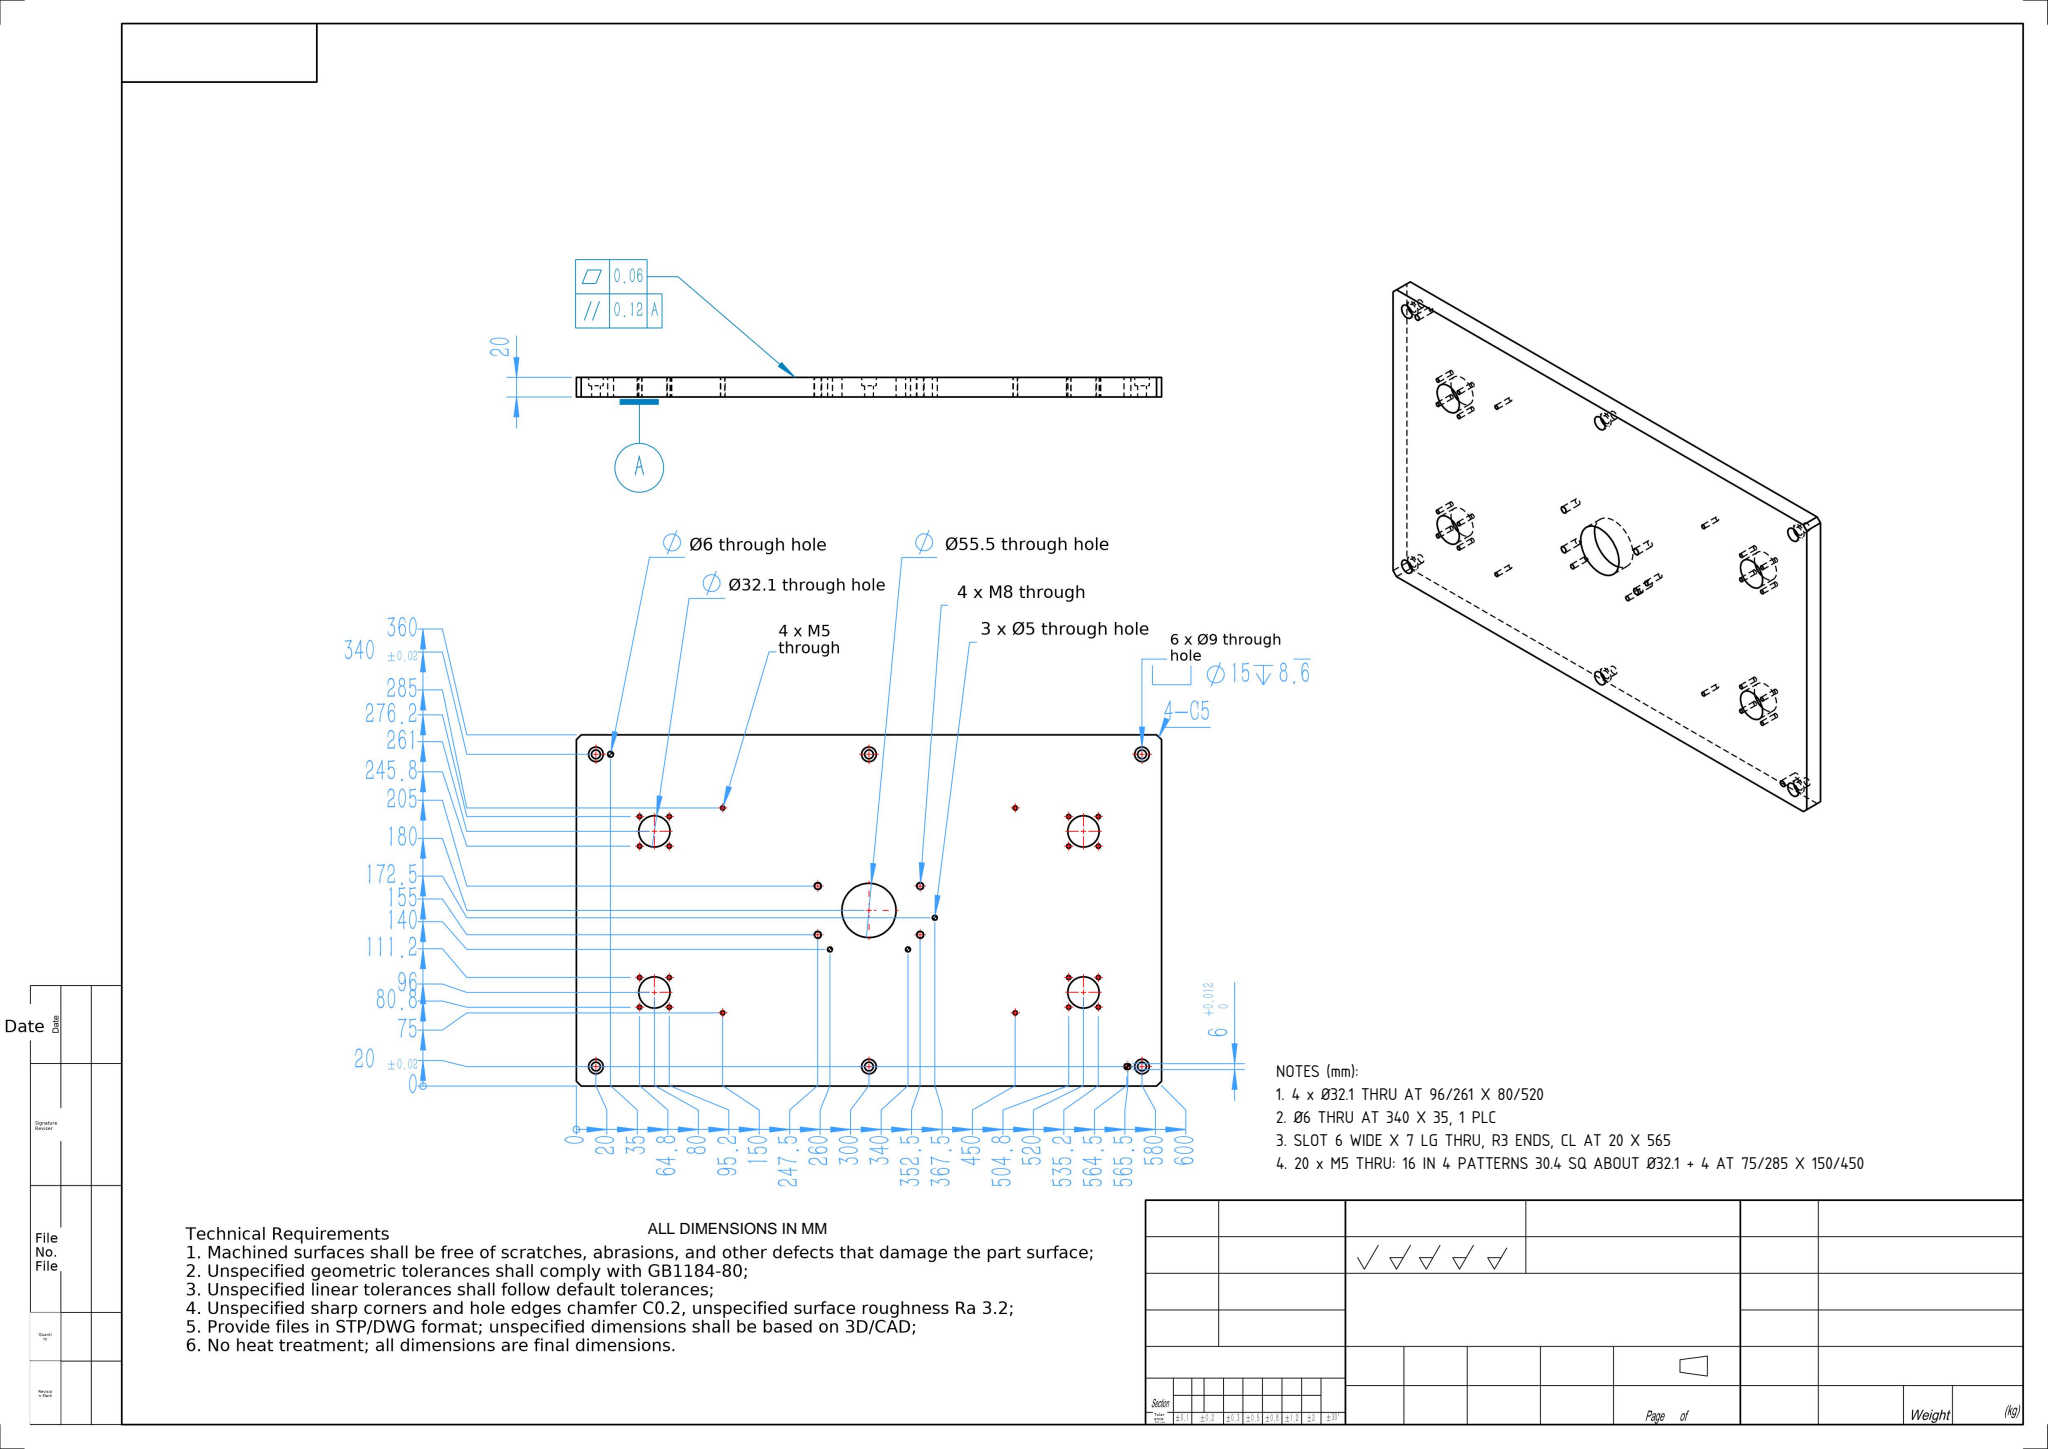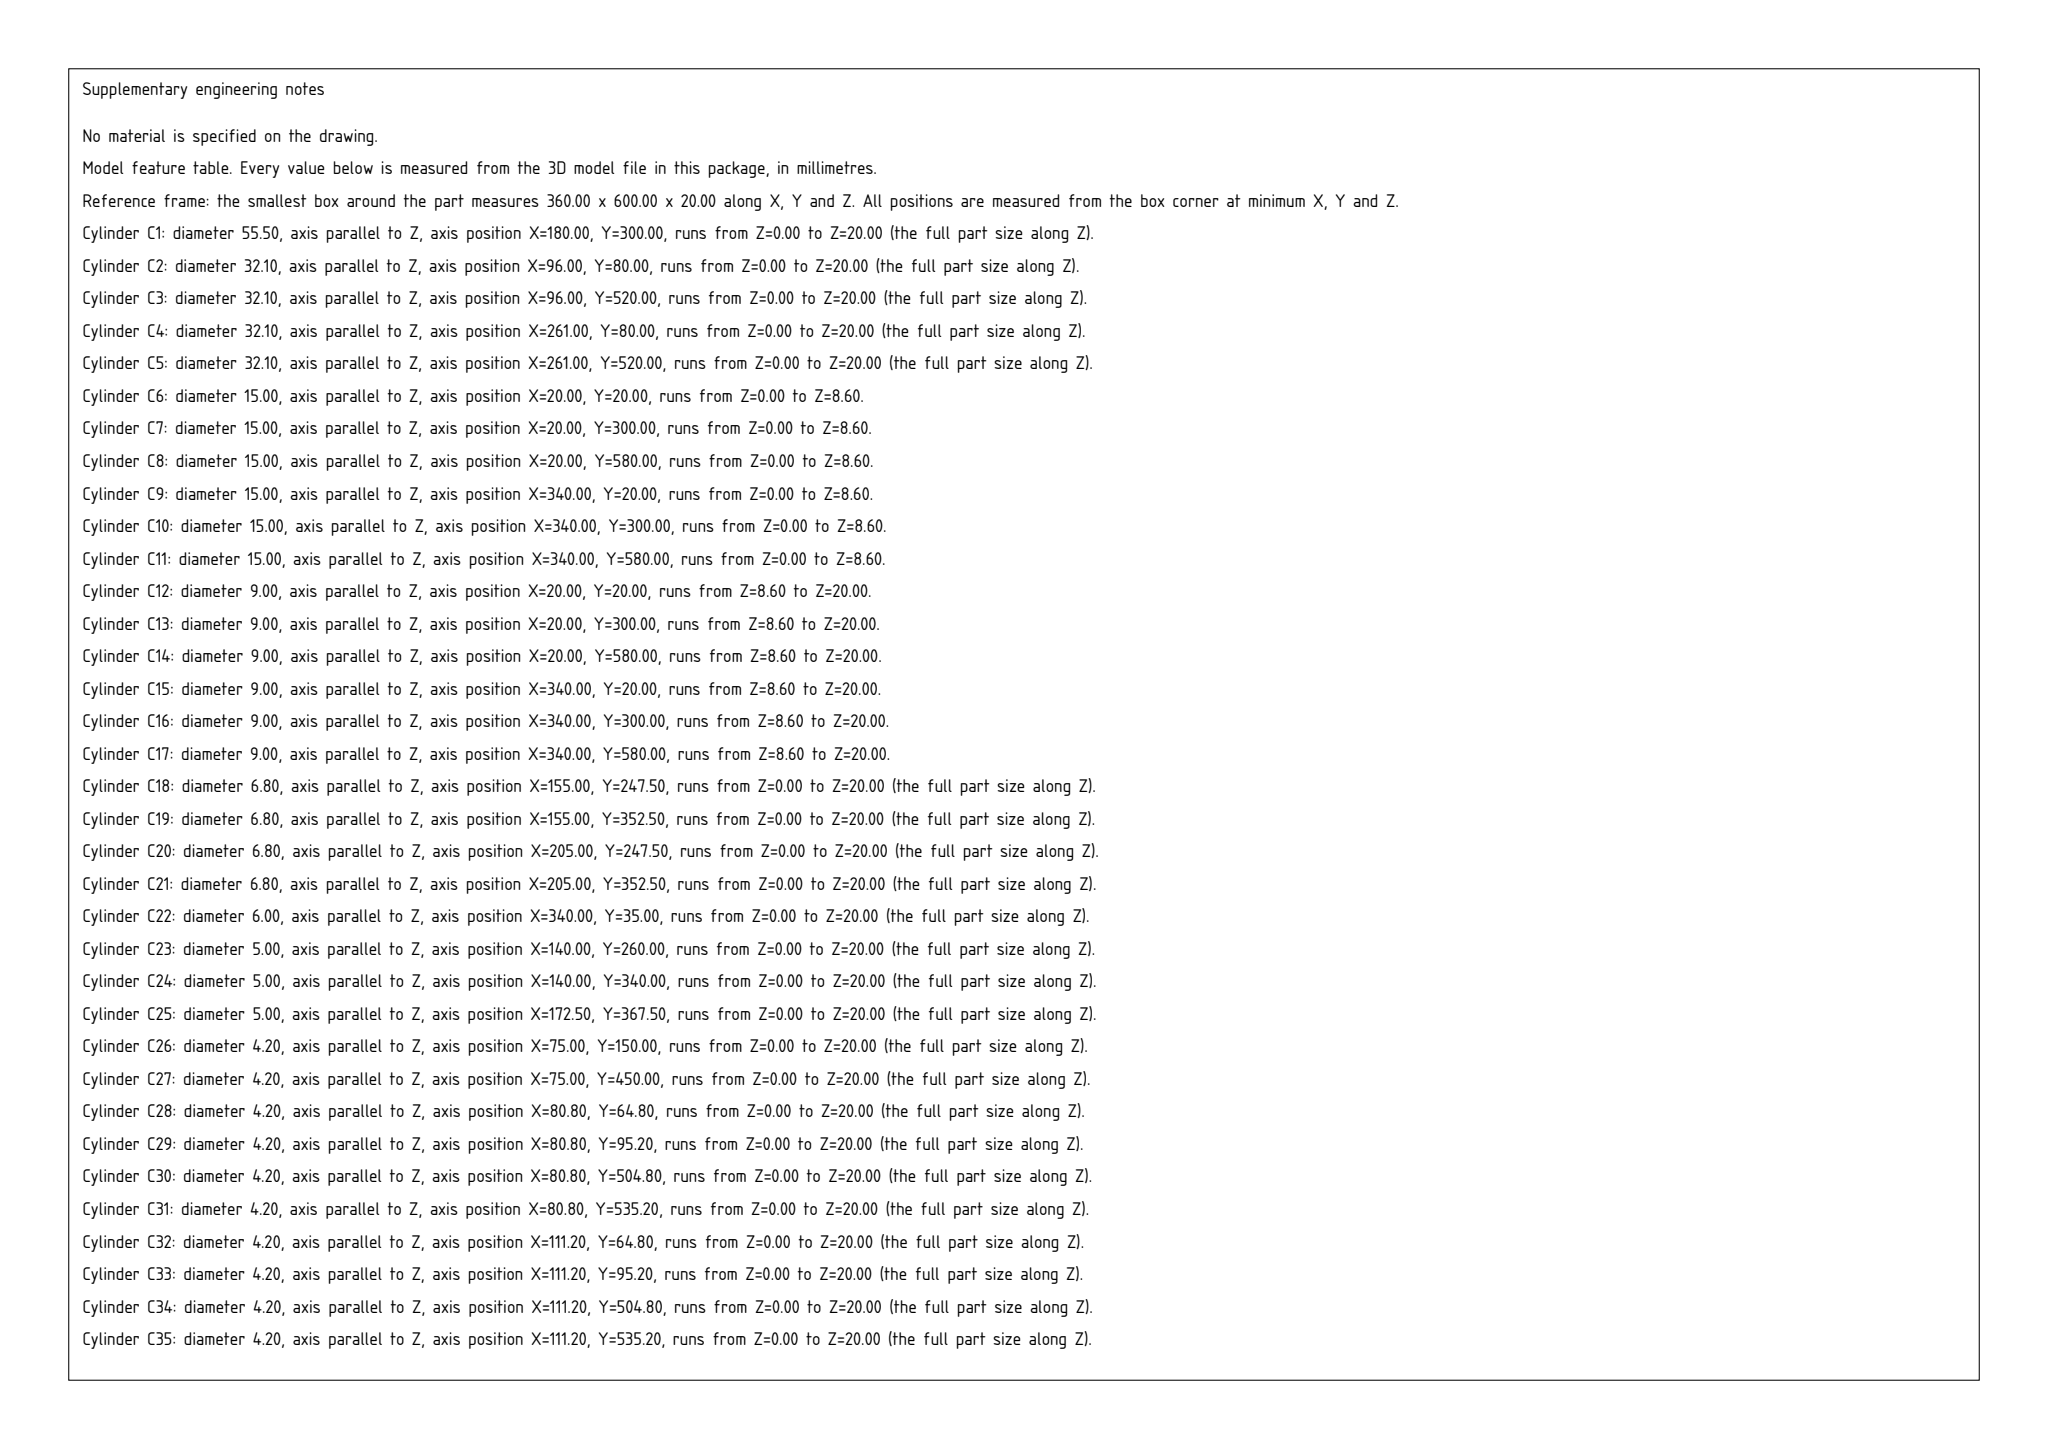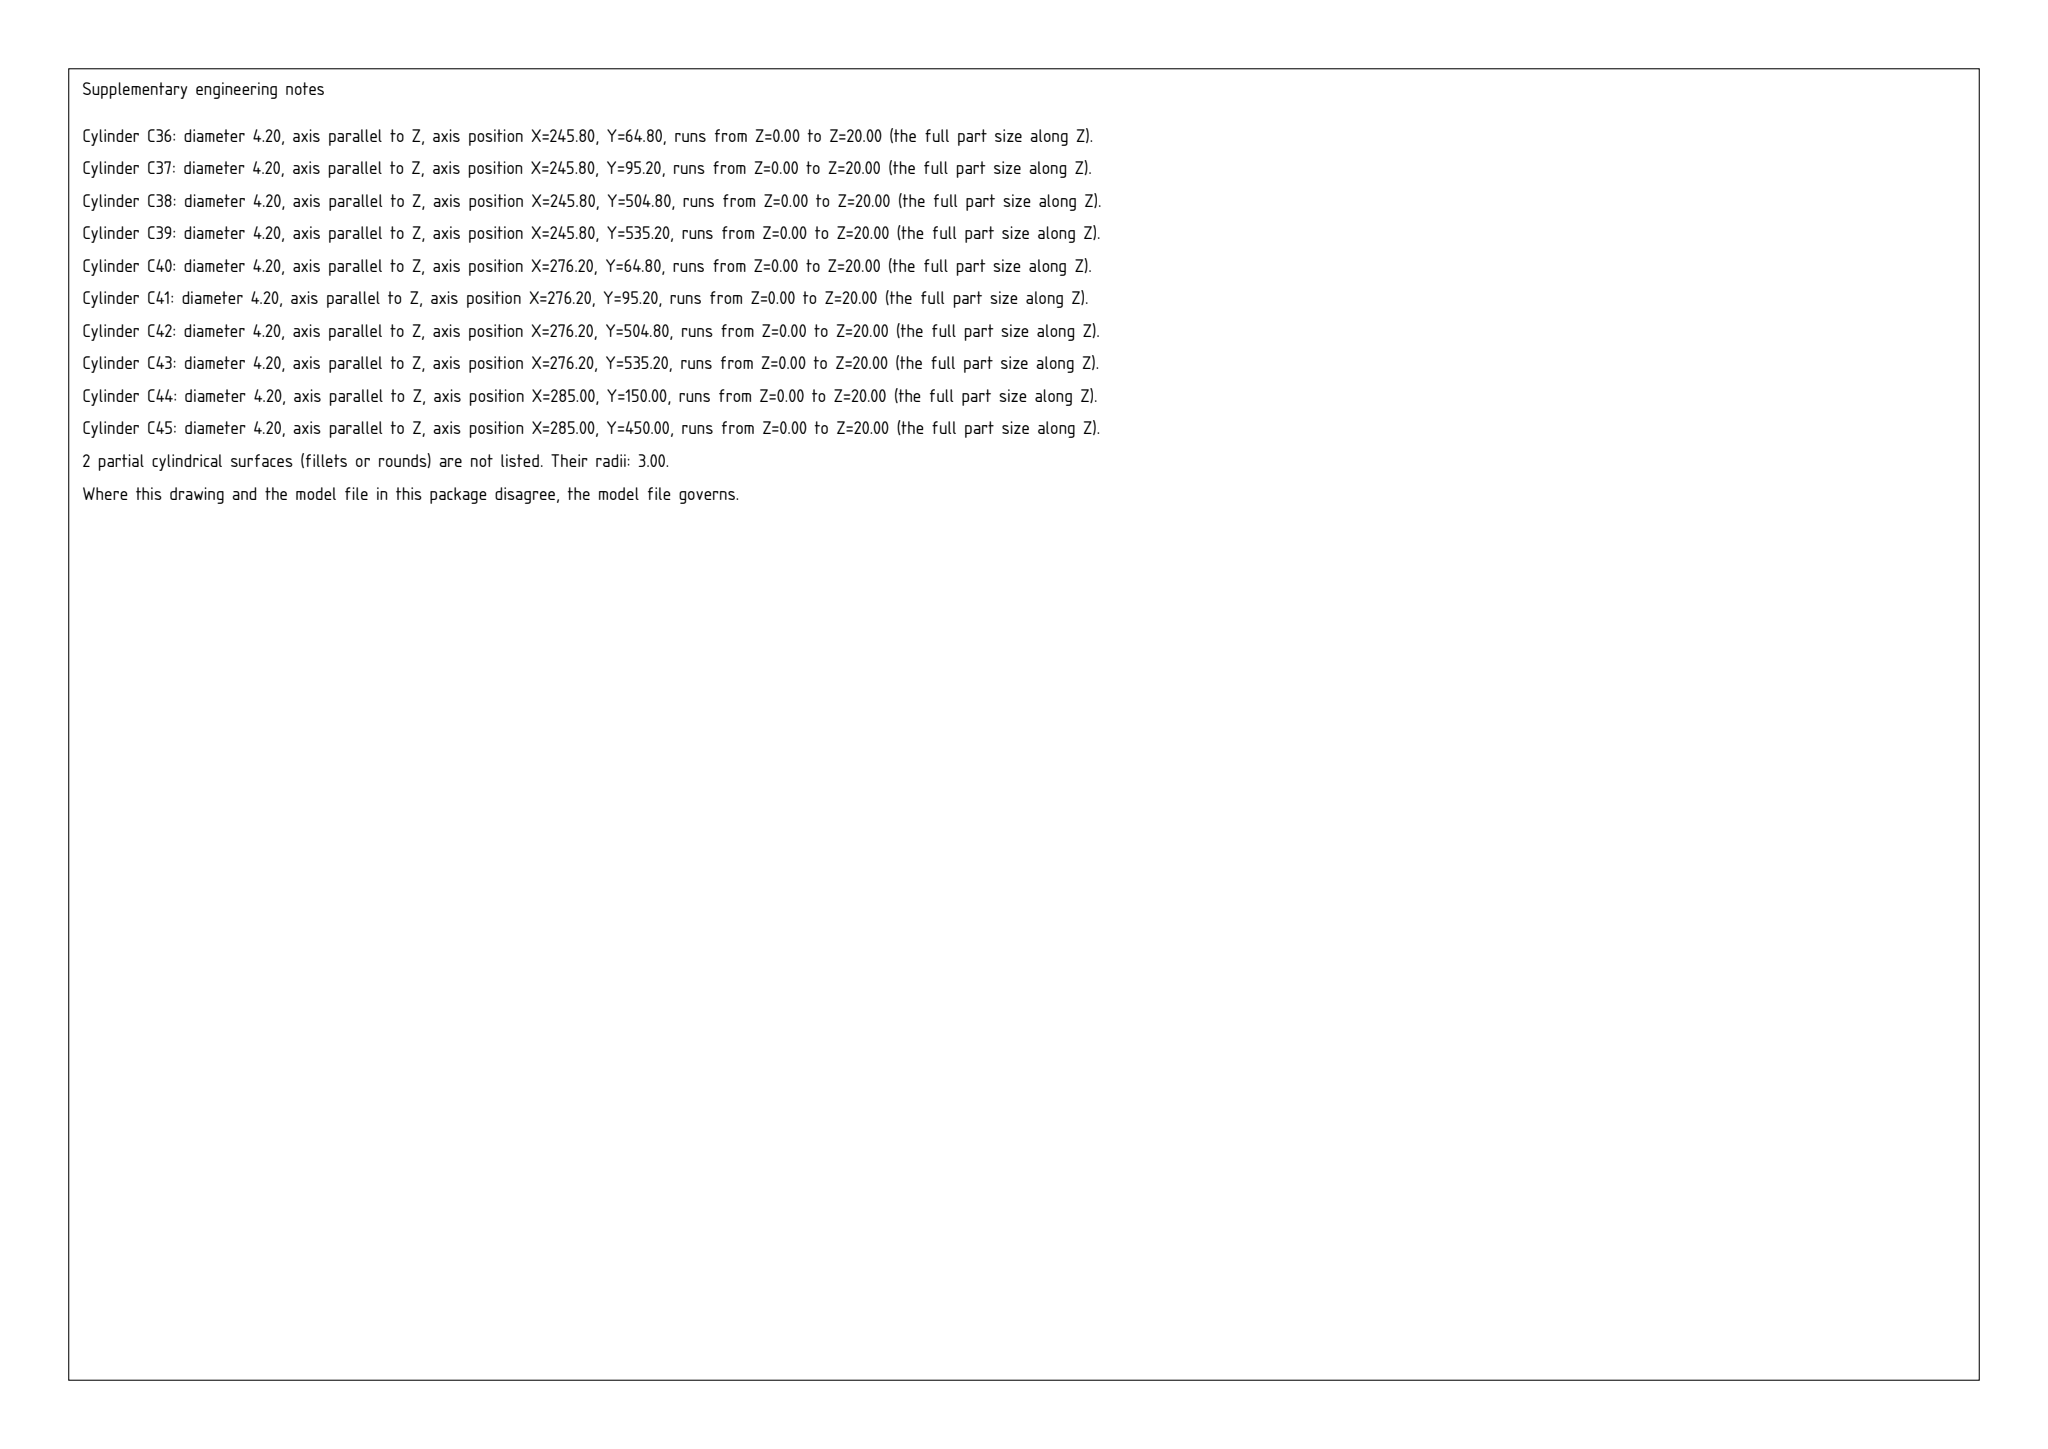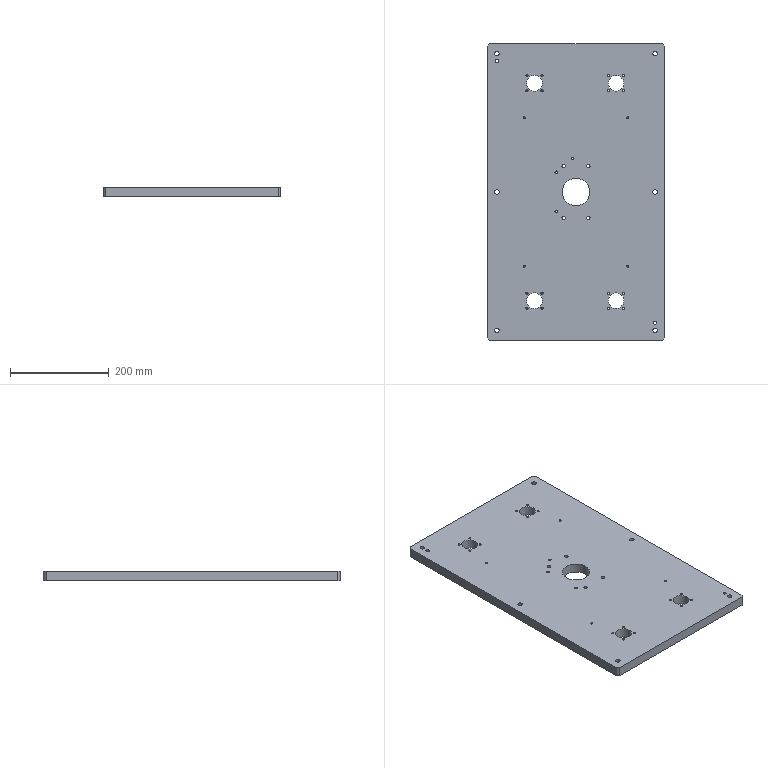Part | SolidWorks | mm | 1 solid | 110 faces | box 360 x 600 x 20 mm | volume 4181527 mm3 | cylinder 92 | plane 18 | commonest cylinder face diameters 4.2 x40 15 x12 9 x12 32.1 x8 6.8 x8 5 x6 6 x4 55.5 x2
Drawing notes:
4 x Ø32.1 THRU AT 96/261 X 80/520 | from the solid: Ø32.1 z thru cyls at (96,80),(96,520),(261,80),(261,520), L=20
Ø6 THRU AT 340 X 35, 1 PLC | from the solid: Single Ø6 z thru cyl at (340,35), L=20
SLOT 6 WIDE X 7 LG THRU, R3 ENDS, CL AT 20 X 565 | from the solid: Two Ø6 thru cyls at (20,564.5) and (20,565.5): obround 6 wide, 7 overall, L=20
20 x M5 THRU: 16 IN 4 PATTERNS 30.4 SQ ABOUT Ø32.1 + 4 AT 75/285 X 150/450 | from the solid: Twenty Ø4.2 thru cyls: 16 at 80.8/111.2/245.8/276.2 x 64.8/95.2/504.8/535.2 (±15.2 about Ø32.1 bores); 4 at (75,150),(75,450),(285,150),(285,450)